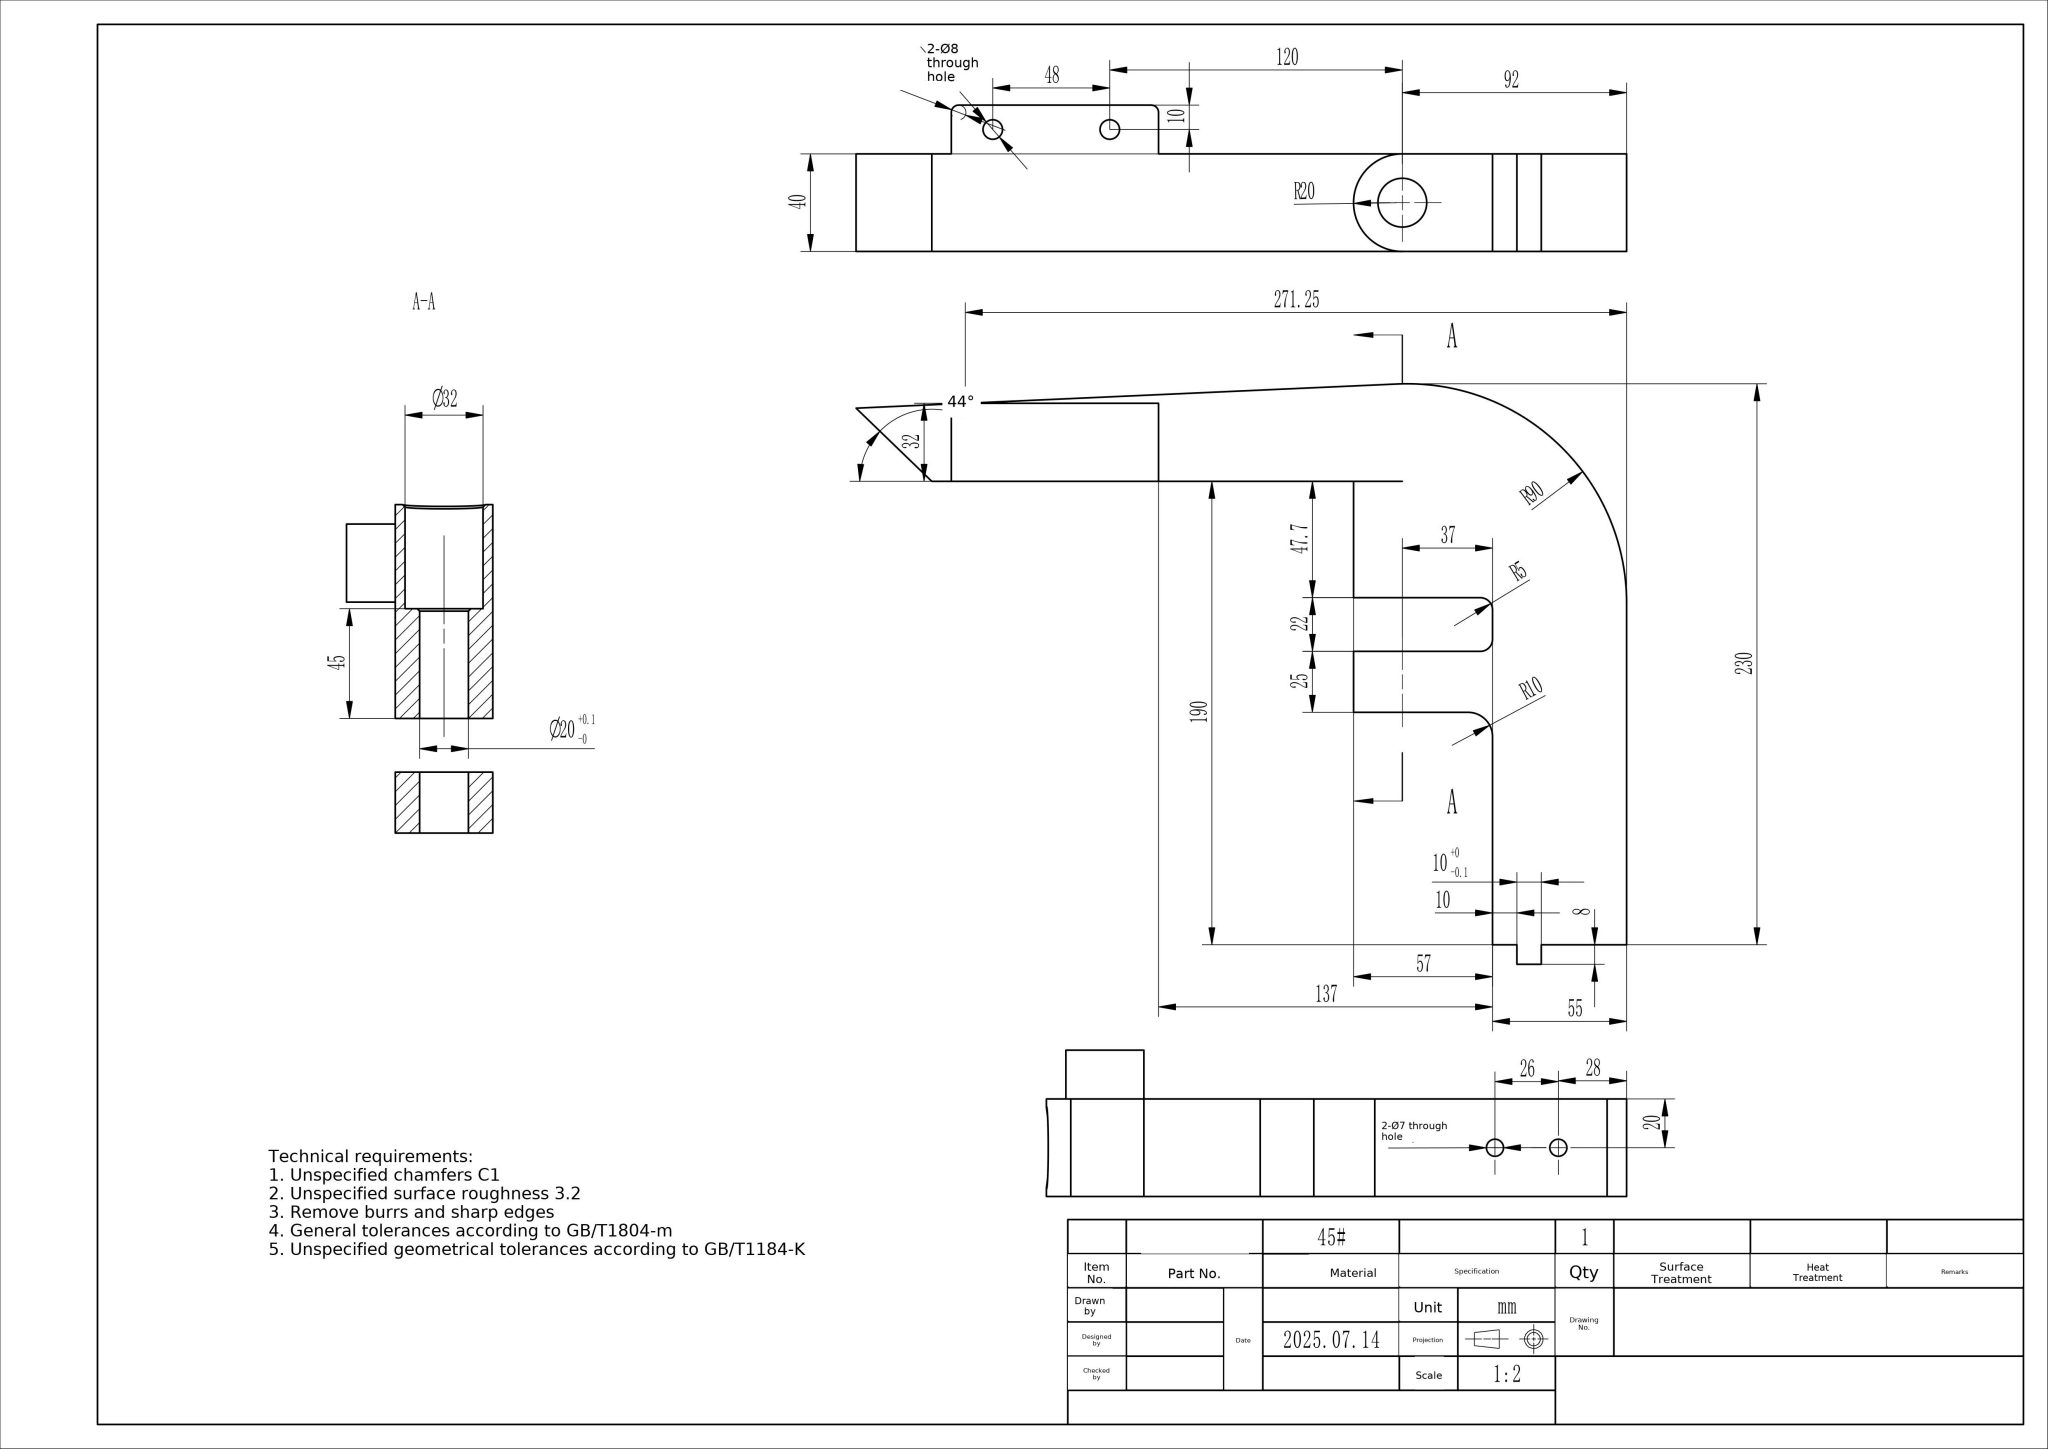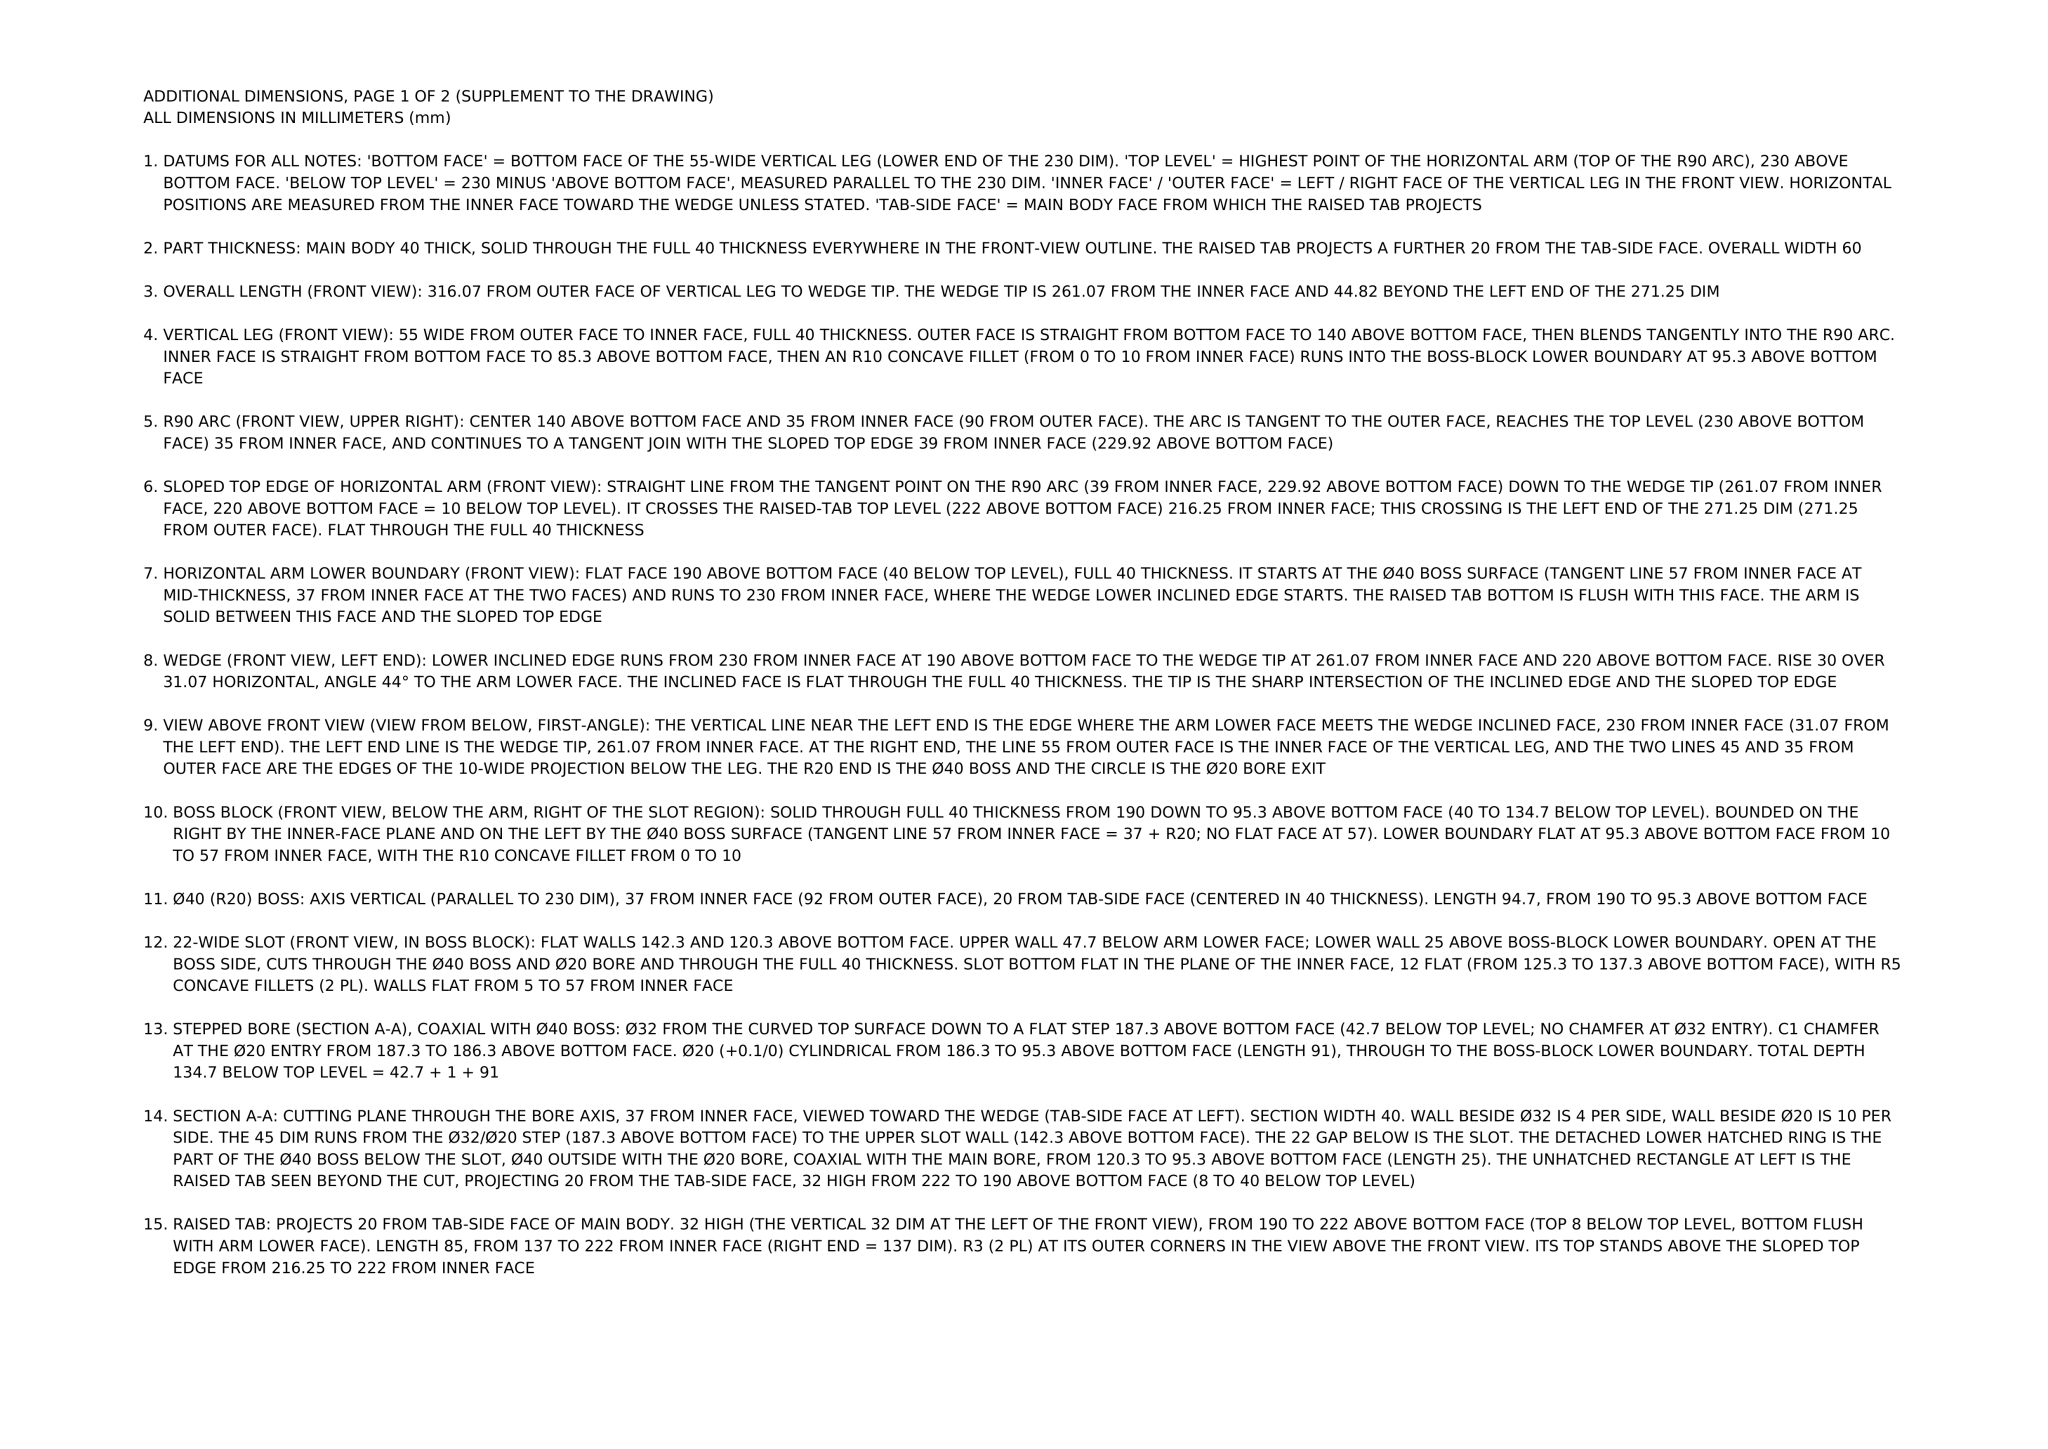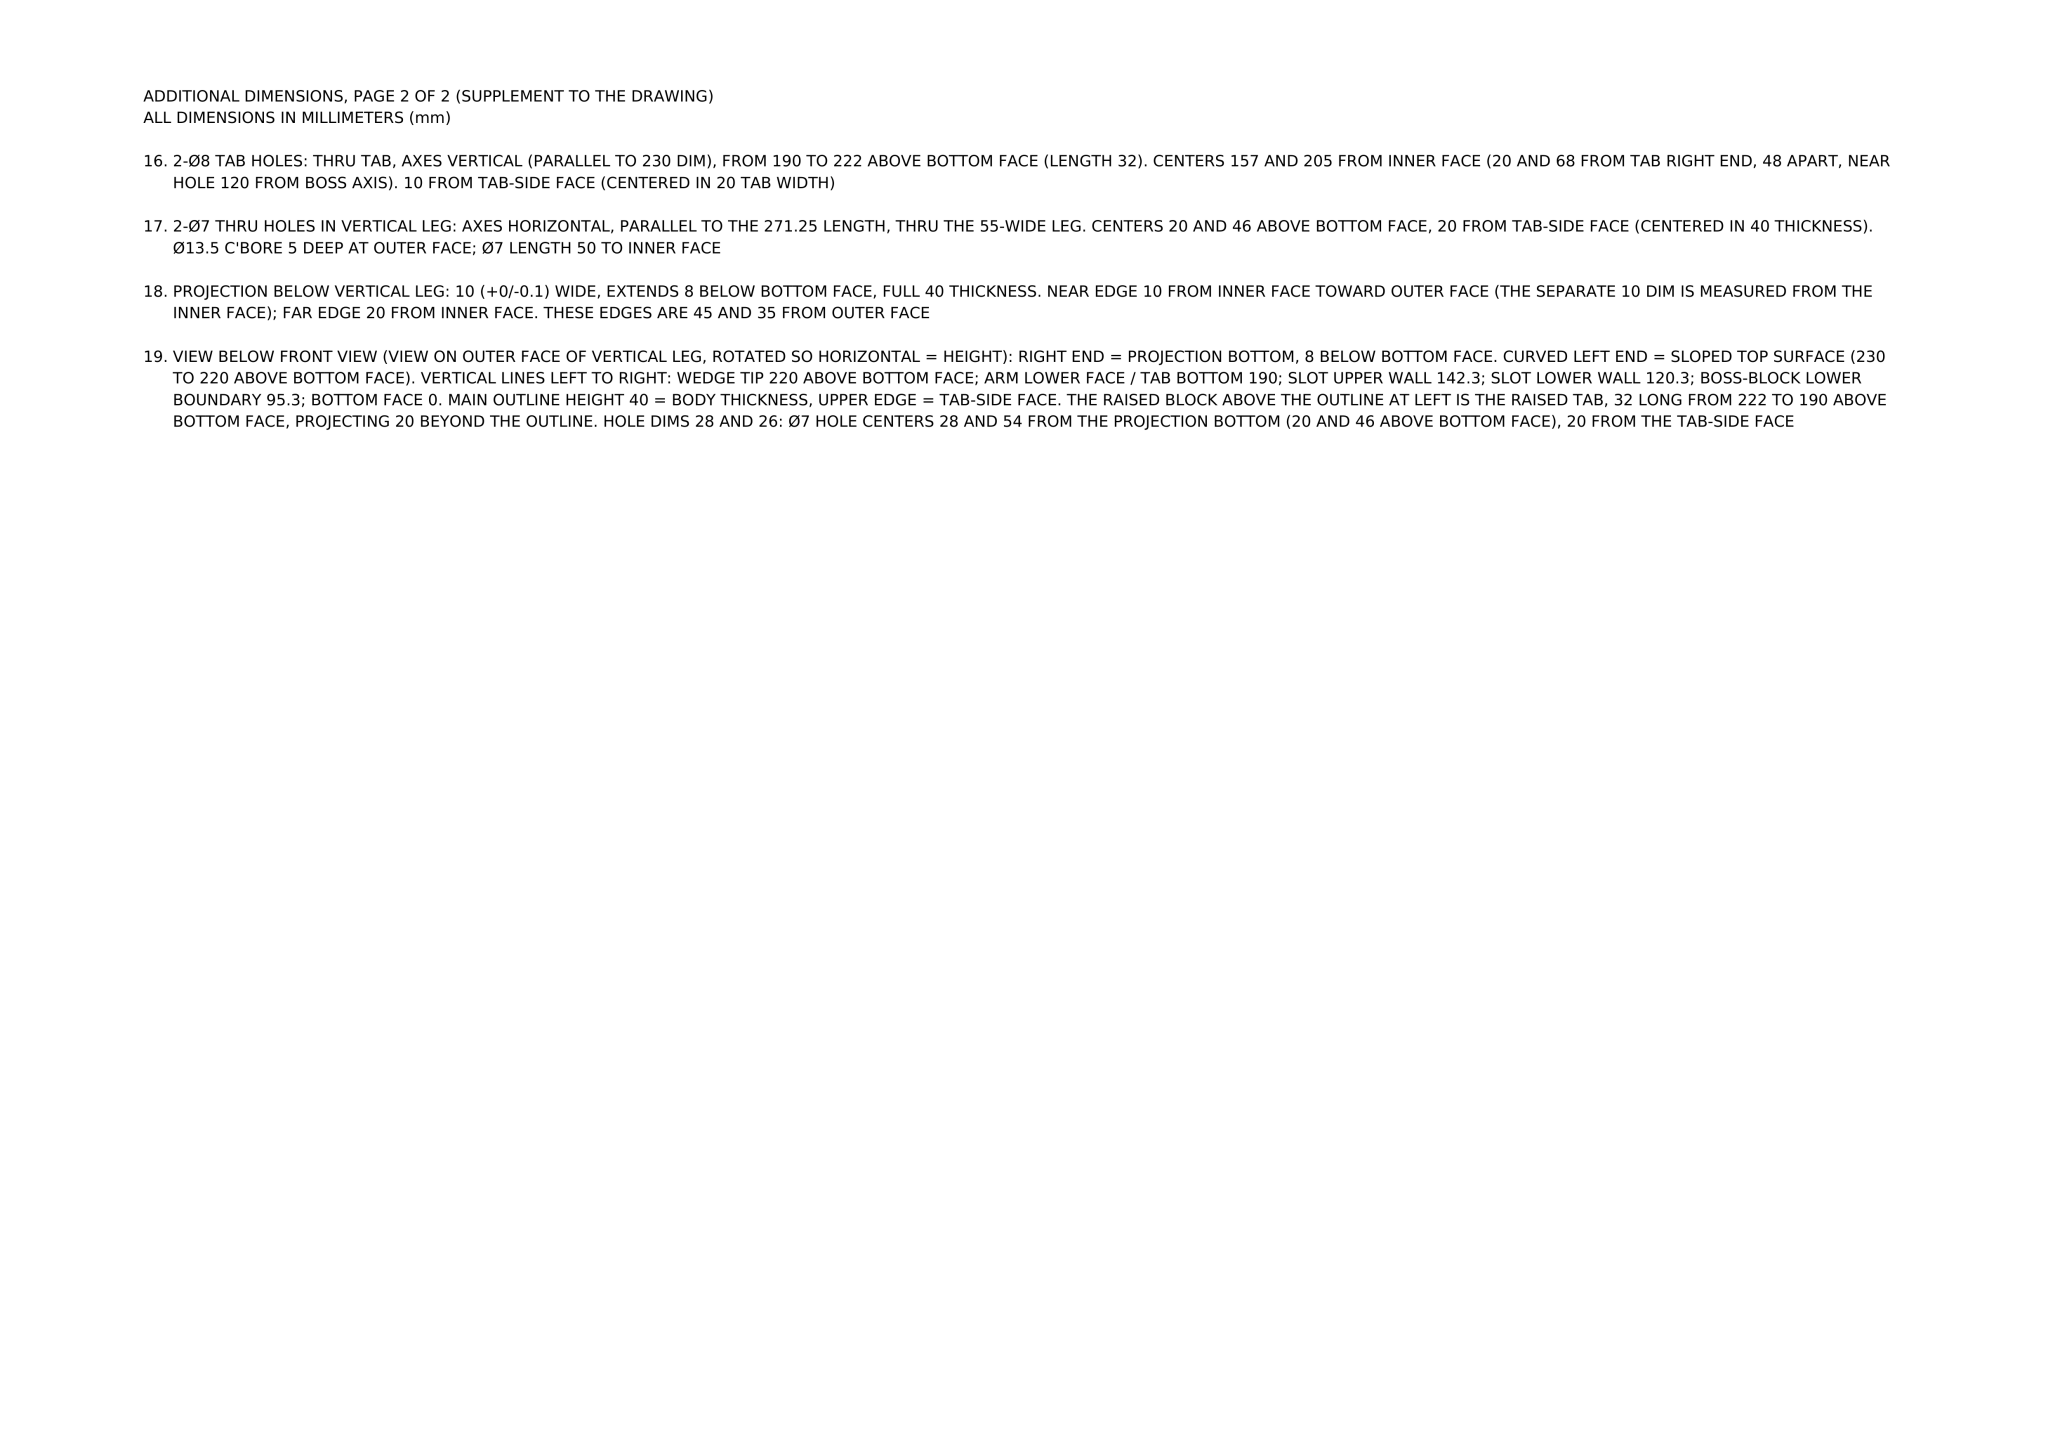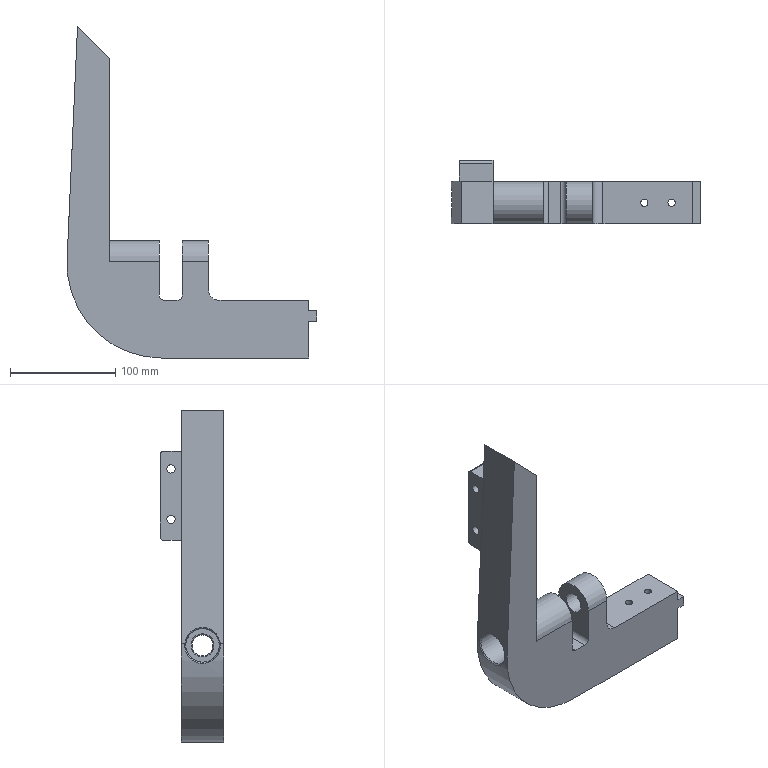Part | NX | mm | 1 solid | 45 faces | box 238 x 60 x 316.07 mm | volume 938077 mm3 | plane 25 | cylinder 17 | spline 2 | cone 1 | commonest cylinder face diameters 20 x3 10 x2 40 x2 7 x2 13.5 x2 8 x2 6 x2 180 x1